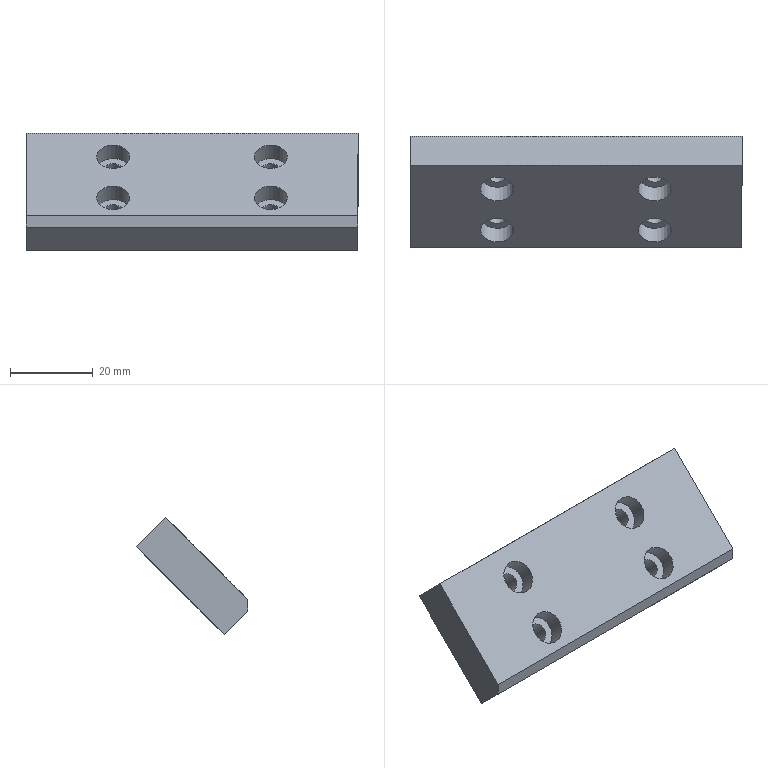Component | SolidWorks | ClampingArm2-1_A27-1 | 1 solid | 27 faces | box 80 x 26.88 x 28.28 mm | volume 22572 mm3 | cylinder 16 | plane 11 | commonest cylinder face diameters 8 x8 4.5 x8 | material Urethane
build123d program:
from build123d import *

# Parameters (mm, degrees)
SKETCH1_W                                          = 80
SKETCH1_H                                          = 30
BOSS_EXTRUDE1_DEPTH                                = 5
HOLE_SIZE_ACCORDING_TO_TYPE_1_OF_HEXAG_D           = 4.5
HOLE_SIZE_ACCORDING_TO_TYPE_1_OF_HEXAG_CBORE_D     = 8
HOLE_SIZE_ACCORDING_TO_TYPE_1_OF_HEXAG_CBORE_DEPTH = 4.6
CHAMFER1_SIZE                                      = 2


with BuildPart() as part:
    # Sketch1 → Boss-Extrude1 (new, symmetric)
    with BuildSketch(Plane(origin=(0, 0, 0), x_dir=(0, 0, -1), z_dir=(1, 0, 0))):
        Rectangle(SKETCH1_W, SKETCH1_H)
    extrude(amount=BOSS_EXTRUDE1_DEPTH, both=True)

    # Hole Size _According to_ Type 1 of Hexag (through all)
    with Locations(Plane(origin=(5, 0, 0), x_dir=(0, 0, -1), z_dir=(1, 0, 0))):
        with Locations((-19, 7), (-19, -7), (19, -7), (19, 7)):
            CounterBoreHole(HOLE_SIZE_ACCORDING_TO_TYPE_1_OF_HEXAG_D / 2, HOLE_SIZE_ACCORDING_TO_TYPE_1_OF_HEXAG_CBORE_D / 2, HOLE_SIZE_ACCORDING_TO_TYPE_1_OF_HEXAG_CBORE_DEPTH)

    # Chamfer1
    chamfer1_edges = [part.edges().sort_by_distance(p)[0] for p in [
        (5, 15, 0),
    ]]
    chamfer(chamfer1_edges, length=CHAMFER1_SIZE)


solid = part.part

# Placed as in the assembly
solid = solid.moved(Location((-43.051, 50.356, -166.066), (-135.019, 90, 0)))
STEP:
#1=CARTESIAN_POINT('',(-0.7894,1.776,-6.722));
#2=VERTEX_POINT('',#1);
#3=CARTESIAN_POINT('',(-1.104,1.776,-6.722));
#4=VERTEX_POINT('',#3);
#5=CARTESIAN_POINT('',(-0.9469,1.776,-6.722));
#6=DIRECTION('',(-0.,-0.7069,0.7073));
#7=DIRECTION('',(-1.,0.,0.));
#8=AXIS2_PLACEMENT_3D('',#5,#6,#7);
#9=CIRCLE('',#8,0.1575);
#10=EDGE_CURVE('',#2,#4,#9,.T.);
#11=ORIENTED_EDGE('',*,*,#10,.F.);
#12=CARTESIAN_POINT('',(-0.7894,1.648,-6.594));
#13=VERTEX_POINT('',#12);
#14=CARTESIAN_POINT('',(-0.7894,1.648,-6.594));
#15=DIRECTION('',(-0.,-0.7069,0.7073));
#16=VECTOR('',#15,39.37);
#17=LINE('',#14,#16);
#18=EDGE_CURVE('',#2,#13,#17,.T.);
#19=ORIENTED_EDGE('',*,*,#18,.T.);
#20=CARTESIAN_POINT('',(-1.104,1.648,-6.594));
#21=VERTEX_POINT('',#20);
#22=CARTESIAN_POINT('',(-0.9469,1.648,-6.594));
#23=DIRECTION('',(-0.,-0.7069,0.7073));
#24=DIRECTION('',(-1.,0.,0.));
#25=AXIS2_PLACEMENT_3D('',#22,#23,#24);
#26=CIRCLE('',#25,0.1575);
#27=EDGE_CURVE('',#13,#21,#26,.T.);
#28=ORIENTED_EDGE('',*,*,#27,.T.);
#29=CARTESIAN_POINT('',(-1.104,1.648,-6.594));
#30=DIRECTION('',(-0.,-0.7069,0.7073));
#31=VECTOR('',#30,39.37);
#32=LINE('',#29,#31);
#33=EDGE_CURVE('',#4,#21,#32,.T.);
#34=ORIENTED_EDGE('',*,*,#33,.F.);
#35=EDGE_LOOP('',(#11,#19,#28,#34));
#36=FACE_OUTER_BOUND('',#35,.T.);
#37=CARTESIAN_POINT('',(-0.9469,1.648,-6.594));
#38=DIRECTION('',(-0.,-0.7069,0.7073));
#39=DIRECTION('',(-1.,0.,0.));
#40=AXIS2_PLACEMENT_3D('',#37,#38,#39);
#41=CYLINDRICAL_SURFACE('',#40,0.1575);
#42=ADVANCED_FACE('',(#36),#41,.F.);
#43=CARTESIAN_POINT('',(-0.8583,1.927,-6.872));
#44=VERTEX_POINT('',#43);
#45=CARTESIAN_POINT('',(-1.035,1.927,-6.872));
#46=VERTEX_POINT('',#45);
#47=CARTESIAN_POINT('',(-0.9469,1.927,-6.872));
#48=DIRECTION('',(-0.,-0.7069,0.7073));
#49=DIRECTION('',(-1.,0.,0.));
#50=AXIS2_PLACEMENT_3D('',#47,#48,#49);
#51=CIRCLE('',#50,0.08858);
#52=EDGE_CURVE('',#44,#46,#51,.T.);
#53=ORIENTED_EDGE('',*,*,#52,.F.);
#54=CARTESIAN_POINT('',(-0.8583,1.776,-6.722));
#55=VERTEX_POINT('',#54);
#56=CARTESIAN_POINT('',(-0.8583,1.648,-6.594));
#57=DIRECTION('',(-0.,-0.7069,0.7073));
#58=VECTOR('',#57,39.37);
#59=LINE('',#56,#58);
#60=EDGE_CURVE('',#44,#55,#59,.T.);
#61=ORIENTED_EDGE('',*,*,#60,.T.);
#62=CARTESIAN_POINT('',(-1.035,1.776,-6.722));
#63=VERTEX_POINT('',#62);
#64=CARTESIAN_POINT('',(-0.9469,1.776,-6.722));
#65=DIRECTION('',(-0.,-0.7069,0.7073));
#66=DIRECTION('',(-1.,0.,0.));
#67=AXIS2_PLACEMENT_3D('',#64,#65,#66);
#68=CIRCLE('',#67,0.08858);
#69=EDGE_CURVE('',#55,#63,#68,.T.);
#70=ORIENTED_EDGE('',*,*,#69,.T.);
#71=CARTESIAN_POINT('',(-1.035,1.648,-6.594));
#72=DIRECTION('',(-0.,-0.7069,0.7073));
#73=VECTOR('',#72,39.37);
#74=LINE('',#71,#73);
#75=EDGE_CURVE('',#46,#63,#74,.T.);
#76=ORIENTED_EDGE('',*,*,#75,.F.);
#77=EDGE_LOOP('',(#53,#61,#70,#76));
#78=FACE_OUTER_BOUND('',#77,.T.);
#79=CARTESIAN_POINT('',(-0.9469,1.648,-6.594));
#80=DIRECTION('',(-0.,-0.7069,0.7073));
#81=DIRECTION('',(-1.,0.,0.));
#82=AXIS2_PLACEMENT_3D('',#79,#80,#81);
#83=CYLINDRICAL_SURFACE('',#82,0.08858);
#84=ADVANCED_FACE('',(#78),#83,.F.);
#85=CARTESIAN_POINT('',(-0.7894,2.166,-6.332));
#86=VERTEX_POINT('',#85);
#87=CARTESIAN_POINT('',(-1.104,2.166,-6.332));
#88=VERTEX_POINT('',#87);
#89=CARTESIAN_POINT('',(-0.9469,2.166,-6.332));
#90=DIRECTION('',(-0.,-0.7069,0.7073));
#91=DIRECTION('',(-1.,0.,0.));
#92=AXIS2_PLACEMENT_3D('',#89,#90,#91);
#93=CIRCLE('',#92,0.1575);
#94=EDGE_CURVE('',#86,#88,#93,.T.);
#95=ORIENTED_EDGE('',*,*,#94,.F.);
#96=CARTESIAN_POINT('',(-0.7894,2.038,-6.204));
#97=VERTEX_POINT('',#96);
#98=CARTESIAN_POINT('',(-0.7894,2.038,-6.204));
#99=DIRECTION('',(-0.,-0.7069,0.7073));
#100=VECTOR('',#99,39.37);
#101=LINE('',#98,#100);
#102=EDGE_CURVE('',#86,#97,#101,.T.);
#103=ORIENTED_EDGE('',*,*,#102,.T.);
#104=CARTESIAN_POINT('',(-1.104,2.038,-6.204));
#105=VERTEX_POINT('',#104);
#106=CARTESIAN_POINT('',(-0.9469,2.038,-6.204));
#107=DIRECTION('',(-0.,-0.7069,0.7073));
#108=DIRECTION('',(-1.,0.,0.));
#109=AXIS2_PLACEMENT_3D('',#106,#107,#108);
#110=CIRCLE('',#109,0.1575);
#111=EDGE_CURVE('',#97,#105,#110,.T.);
#112=ORIENTED_EDGE('',*,*,#111,.T.);
#113=CARTESIAN_POINT('',(-1.104,2.038,-6.204));
#114=DIRECTION('',(-0.,-0.7069,0.7073));
#115=VECTOR('',#114,39.37);
#116=LINE('',#113,#115);
#117=EDGE_CURVE('',#88,#105,#116,.T.);
#118=ORIENTED_EDGE('',*,*,#117,.F.);
#119=EDGE_LOOP('',(#95,#103,#112,#118));
#120=FACE_OUTER_BOUND('',#119,.T.);
#121=CARTESIAN_POINT('',(-0.9469,2.038,-6.204));
#122=DIRECTION('',(-0.,-0.7069,0.7073));
#123=DIRECTION('',(-1.,0.,0.));
#124=AXIS2_PLACEMENT_3D('',#121,#122,#123);
#125=CYLINDRICAL_SURFACE('',#124,0.1575);
#126=ADVANCED_FACE('',(#120),#125,.F.);
#127=CARTESIAN_POINT('',(-0.8583,2.317,-6.482));
#128=VERTEX_POINT('',#127);
#129=CARTESIAN_POINT('',(-1.035,2.317,-6.482));
#130=VERTEX_POINT('',#129);
#131=CARTESIAN_POINT('',(-0.9469,2.317,-6.482));
#132=DIRECTION('',(-0.,-0.7069,0.7073));
#133=DIRECTION('',(-1.,0.,0.));
#134=AXIS2_PLACEMENT_3D('',#131,#132,#133);
#135=CIRCLE('',#134,0.08858);
#136=EDGE_CURVE('',#128,#130,#135,.T.);
#137=ORIENTED_EDGE('',*,*,#136,.F.);
#138=CARTESIAN_POINT('',(-0.8583,2.166,-6.332));
#139=VERTEX_POINT('',#138);
#140=CARTESIAN_POINT('',(-0.8583,2.038,-6.204));
#141=DIRECTION('',(-0.,-0.7069,0.7073));
#142=VECTOR('',#141,39.37);
#143=LINE('',#140,#142);
#144=EDGE_CURVE('',#128,#139,#143,.T.);
#145=ORIENTED_EDGE('',*,*,#144,.T.);
#146=CARTESIAN_POINT('',(-1.035,2.166,-6.332));
#147=VERTEX_POINT('',#146);
#148=CARTESIAN_POINT('',(-0.9469,2.166,-6.332));
#149=DIRECTION('',(-0.,-0.7069,0.7073));
#150=DIRECTION('',(-1.,0.,0.));
#151=AXIS2_PLACEMENT_3D('',#148,#149,#150);
#152=CIRCLE('',#151,0.08858);
#153=EDGE_CURVE('',#139,#147,#152,.T.);
#154=ORIENTED_EDGE('',*,*,#153,.T.);
#155=CARTESIAN_POINT('',(-1.035,2.038,-6.204));
#156=DIRECTION('',(-0.,-0.7069,0.7073));
#157=VECTOR('',#156,39.37);
#158=LINE('',#155,#157);
#159=EDGE_CURVE('',#130,#147,#158,.T.);
#160=ORIENTED_EDGE('',*,*,#159,.F.);
#161=EDGE_LOOP('',(#137,#145,#154,#160));
#162=FACE_OUTER_BOUND('',#161,.T.);
#163=CARTESIAN_POINT('',(-0.9469,2.038,-6.204));
#164=DIRECTION('',(-0.,-0.7069,0.7073));
#165=DIRECTION('',(-1.,0.,0.));
#166=AXIS2_PLACEMENT_3D('',#163,#164,#165);
#167=CYLINDRICAL_SURFACE('',#166,0.08858);
#168=ADVANCED_FACE('',(#162),#167,.F.);
#169=CARTESIAN_POINT('',(-2.285,2.166,-6.332));
#170=VERTEX_POINT('',#169);
#171=CARTESIAN_POINT('',(-2.6,2.166,-6.332));
#172=VERTEX_POINT('',#171);
#173=CARTESIAN_POINT('',(-2.443,2.166,-6.332));
#174=DIRECTION('',(-0.,-0.7069,0.7073));
#175=DIRECTION('',(-1.,0.,0.));
#176=AXIS2_PLACEMENT_3D('',#173,#174,#175);
#177=CIRCLE('',#176,0.1575);
#178=EDGE_CURVE('',#170,#172,#177,.T.);
#179=ORIENTED_EDGE('',*,*,#178,.F.);
#180=CARTESIAN_POINT('',(-2.285,2.038,-6.204));
#181=VERTEX_POINT('',#180);
#182=CARTESIAN_POINT('',(-2.285,2.038,-6.204));
#183=DIRECTION('',(-0.,-0.7069,0.7073));
#184=VECTOR('',#183,39.37);
#185=LINE('',#182,#184);
#186=EDGE_CURVE('',#170,#181,#185,.T.);
#187=ORIENTED_EDGE('',*,*,#186,.T.);
#188=CARTESIAN_POINT('',(-2.6,2.038,-6.204));
#189=VERTEX_POINT('',#188);
#190=CARTESIAN_POINT('',(-2.443,2.038,-6.204));
#191=DIRECTION('',(-0.,-0.7069,0.7073));
#192=DIRECTION('',(-1.,0.,0.));
#193=AXIS2_PLACEMENT_3D('',#190,#191,#192);
#194=CIRCLE('',#193,0.1575);
#195=EDGE_CURVE('',#181,#189,#194,.T.);
#196=ORIENTED_EDGE('',*,*,#195,.T.);
#197=CARTESIAN_POINT('',(-2.6,2.038,-6.204));
#198=DIRECTION('',(-0.,-0.7069,0.7073));
#199=VECTOR('',#198,39.37);
#200=LINE('',#197,#199);
#201=EDGE_CURVE('',#172,#189,#200,.T.);
#202=ORIENTED_EDGE('',*,*,#201,.F.);
#203=EDGE_LOOP('',(#179,#187,#196,#202));
#204=FACE_OUTER_BOUND('',#203,.T.);
#205=CARTESIAN_POINT('',(-2.443,2.038,-6.204));
#206=DIRECTION('',(-0.,-0.7069,0.7073));
#207=DIRECTION('',(-1.,0.,0.));
#208=AXIS2_PLACEMENT_3D('',#205,#206,#207);
#209=CYLINDRICAL_SURFACE('',#208,0.1575);
#210=ADVANCED_FACE('',(#204),#209,.F.);
#211=CARTESIAN_POINT('',(-2.354,2.317,-6.482));
#212=VERTEX_POINT('',#211);
#213=CARTESIAN_POINT('',(-2.532,2.317,-6.482));
#214=VERTEX_POINT('',#213);
#215=CARTESIAN_POINT('',(-2.443,2.317,-6.482));
#216=DIRECTION('',(-0.,-0.7069,0.7073));
#217=DIRECTION('',(-1.,0.,0.));
#218=AXIS2_PLACEMENT_3D('',#215,#216,#217);
#219=CIRCLE('',#218,0.08858);
#220=EDGE_CURVE('',#212,#214,#219,.T.);
#221=ORIENTED_EDGE('',*,*,#220,.F.);
#222=CARTESIAN_POINT('',(-2.354,2.166,-6.332));
#223=VERTEX_POINT('',#222);
#224=CARTESIAN_POINT('',(-2.354,2.038,-6.204));
#225=DIRECTION('',(-0.,-0.7069,0.7073));
#226=VECTOR('',#225,39.37);
#227=LINE('',#224,#226);
#228=EDGE_CURVE('',#212,#223,#227,.T.);
#229=ORIENTED_EDGE('',*,*,#228,.T.);
#230=CARTESIAN_POINT('',(-2.532,2.166,-6.332));
#231=VERTEX_POINT('',#230);
#232=CARTESIAN_POINT('',(-2.443,2.166,-6.332));
#233=DIRECTION('',(-0.,-0.7069,0.7073));
#234=DIRECTION('',(-1.,0.,0.));
#235=AXIS2_PLACEMENT_3D('',#232,#233,#234);
#236=CIRCLE('',#235,0.08858);
#237=EDGE_CURVE('',#223,#231,#236,.T.);
#238=ORIENTED_EDGE('',*,*,#237,.T.);
#239=CARTESIAN_POINT('',(-2.532,2.038,-6.204));
#240=DIRECTION('',(-0.,-0.7069,0.7073));
#241=VECTOR('',#240,39.37);
#242=LINE('',#239,#241);
#243=EDGE_CURVE('',#214,#231,#242,.T.);
#244=ORIENTED_EDGE('',*,*,#243,.F.);
#245=EDGE_LOOP('',(#221,#229,#238,#244));
#246=FACE_OUTER_BOUND('',#245,.T.);
#247=CARTESIAN_POINT('',(-2.443,2.038,-6.204));
#248=DIRECTION('',(-0.,-0.7069,0.7073));
#249=DIRECTION('',(-1.,0.,0.));
#250=AXIS2_PLACEMENT_3D('',#247,#248,#249);
#251=CYLINDRICAL_SURFACE('',#250,0.08858);
#252=ADVANCED_FACE('',(#246),#251,.F.);
#253=CARTESIAN_POINT('',(-2.285,1.776,-6.722));
#254=VERTEX_POINT('',#253);
#255=CARTESIAN_POINT('',(-2.6,1.776,-6.722));
#256=VERTEX_POINT('',#255);
#257=CARTESIAN_POINT('',(-2.443,1.776,-6.722));
#258=DIRECTION('',(-0.,-0.7069,0.7073));
#259=DIRECTION('',(-1.,0.,0.));
#260=AXIS2_PLACEMENT_3D('',#257,#258,#259);
#261=CIRCLE('',#260,0.1575);
#262=EDGE_CURVE('',#254,#256,#261,.T.);
#263=ORIENTED_EDGE('',*,*,#262,.F.);
#264=CARTESIAN_POINT('',(-2.285,1.648,-6.594));
#265=VERTEX_POINT('',#264);
#266=CARTESIAN_POINT('',(-2.285,1.648,-6.594));
#267=DIRECTION('',(-0.,-0.7069,0.7073));
#268=VECTOR('',#267,39.37);
#269=LINE('',#266,#268);
#270=EDGE_CURVE('',#254,#265,#269,.T.);
#271=ORIENTED_EDGE('',*,*,#270,.T.);
#272=CARTESIAN_POINT('',(-2.6,1.648,-6.594));
#273=VERTEX_POINT('',#272);
#274=CARTESIAN_POINT('',(-2.443,1.648,-6.594));
#275=DIRECTION('',(-0.,-0.7069,0.7073));
#276=DIRECTION('',(-1.,0.,0.));
#277=AXIS2_PLACEMENT_3D('',#274,#275,#276);
#278=CIRCLE('',#277,0.1575);
#279=EDGE_CURVE('',#265,#273,#278,.T.);
#280=ORIENTED_EDGE('',*,*,#279,.T.);
#281=CARTESIAN_POINT('',(-2.6,1.648,-6.594));
#282=DIRECTION('',(-0.,-0.7069,0.7073));
#283=VECTOR('',#282,39.37);
#284=LINE('',#281,#283);
#285=EDGE_CURVE('',#256,#273,#284,.T.);
#286=ORIENTED_EDGE('',*,*,#285,.F.);
#287=EDGE_LOOP('',(#263,#271,#280,#286));
#288=FACE_OUTER_BOUND('',#287,.T.);
#289=CARTESIAN_POINT('',(-2.443,1.648,-6.594));
#290=DIRECTION('',(-0.,-0.7069,0.7073));
#291=DIRECTION('',(-1.,0.,0.));
#292=AXIS2_PLACEMENT_3D('',#289,#290,#291);
#293=CYLINDRICAL_SURFACE('',#292,0.1575);
#294=ADVANCED_FACE('',(#288),#293,.F.);
#295=CARTESIAN_POINT('',(-2.354,1.927,-6.872));
#296=VERTEX_POINT('',#295);
#297=CARTESIAN_POINT('',(-2.532,1.927,-6.872));
#298=VERTEX_POINT('',#297);
#299=CARTESIAN_POINT('',(-2.443,1.927,-6.872));
#300=DIRECTION('',(-0.,-0.7069,0.7073));
#301=DIRECTION('',(-1.,0.,0.));
#302=AXIS2_PLACEMENT_3D('',#299,#300,#301);
#303=CIRCLE('',#302,0.08858);
#304=EDGE_CURVE('',#296,#298,#303,.T.);
#305=ORIENTED_EDGE('',*,*,#304,.F.);
#306=CARTESIAN_POINT('',(-2.354,1.776,-6.722));
#307=VERTEX_POINT('',#306);
#308=CARTESIAN_POINT('',(-2.354,1.648,-6.594));
#309=DIRECTION('',(-0.,-0.7069,0.7073));
#310=VECTOR('',#309,39.37);
#311=LINE('',#308,#310);
#312=EDGE_CURVE('',#296,#307,#311,.T.);
#313=ORIENTED_EDGE('',*,*,#312,.T.);
#314=CARTESIAN_POINT('',(-2.532,1.776,-6.722));
#315=VERTEX_POINT('',#314);
#316=CARTESIAN_POINT('',(-2.443,1.776,-6.722));
#317=DIRECTION('',(-0.,-0.7069,0.7073));
#318=DIRECTION('',(-1.,0.,0.));
#319=AXIS2_PLACEMENT_3D('',#316,#317,#318);
#320=CIRCLE('',#319,0.08858);
#321=EDGE_CURVE('',#307,#315,#320,.T.);
#322=ORIENTED_EDGE('',*,*,#321,.T.);
#323=CARTESIAN_POINT('',(-2.532,1.648,-6.594));
#324=DIRECTION('',(-0.,-0.7069,0.7073));
#325=VECTOR('',#324,39.37);
#326=LINE('',#323,#325);
#327=EDGE_CURVE('',#298,#315,#326,.T.);
#328=ORIENTED_EDGE('',*,*,#327,.F.);
#329=EDGE_LOOP('',(#305,#313,#322,#328));
#330=FACE_OUTER_BOUND('',#329,.T.);
#331=CARTESIAN_POINT('',(-2.443,1.648,-6.594));
#332=DIRECTION('',(-0.,-0.7069,0.7073));
#333=DIRECTION('',(-1.,0.,0.));
#334=AXIS2_PLACEMENT_3D('',#331,#332,#333);
#335=CYLINDRICAL_SURFACE('',#334,0.08858);
#336=ADVANCED_FACE('',(#330),#335,.F.);
#337=CARTESIAN_POINT('',(-3.27,1.481,-6.872));
#338=VERTEX_POINT('',#337);
#339=CARTESIAN_POINT('',(-3.27,1.704,-7.095));
#340=VERTEX_POINT('',#339);
#341=CARTESIAN_POINT('',(-3.27,1.426,-6.816));
#342=DIRECTION('',(0.,0.7069,-0.7073));
#343=VECTOR('',#342,39.37);
#344=LINE('',#341,#343);
#345=EDGE_CURVE('',#338,#340,#344,.T.);
#346=ORIENTED_EDGE('',*,*,#345,.F.);
#347=CARTESIAN_POINT('',(-3.27,1.481,-6.761));
#348=VERTEX_POINT('',#347);
#349=CARTESIAN_POINT('',(-3.27,1.481,-6.761));
#350=DIRECTION('',(0.,0.0003333,1.));
#351=VECTOR('',#350,39.37);
#352=LINE('',#349,#351);
#353=EDGE_CURVE('',#338,#348,#352,.T.);
#354=ORIENTED_EDGE('',*,*,#353,.T.);
#355=CARTESIAN_POINT('',(-3.27,2.261,-5.981));
#356=VERTEX_POINT('',#355);
#357=CARTESIAN_POINT('',(-3.27,1.426,-6.816));
#358=DIRECTION('',(-0.,-0.7073,-0.7069));
#359=VECTOR('',#358,39.37);
#360=LINE('',#357,#359);
#361=EDGE_CURVE('',#356,#348,#360,.T.);
#362=ORIENTED_EDGE('',*,*,#361,.F.);
#363=CARTESIAN_POINT('',(-3.27,2.539,-6.26));
#364=VERTEX_POINT('',#363);
#365=CARTESIAN_POINT('',(-3.27,2.261,-5.981));
#366=DIRECTION('',(0.,0.7069,-0.7073));
#367=VECTOR('',#366,39.37);
#368=LINE('',#365,#367);
#369=EDGE_CURVE('',#356,#364,#368,.T.);
#370=ORIENTED_EDGE('',*,*,#369,.T.);
#371=CARTESIAN_POINT('',(-3.27,1.704,-7.095));
#372=DIRECTION('',(-0.,-0.7073,-0.7069));
#373=VECTOR('',#372,39.37);
#374=LINE('',#371,#373);
#375=EDGE_CURVE('',#364,#340,#374,.T.);
#376=ORIENTED_EDGE('',*,*,#375,.T.);
#377=EDGE_LOOP('',(#346,#354,#362,#370,#376));
#378=FACE_OUTER_BOUND('',#377,.T.);
#379=CARTESIAN_POINT('',(-3.27,1.426,-6.816));
#380=DIRECTION('',(1.,-0.,-0.));
#381=DIRECTION('',(0.,0.7073,0.7069));
#382=AXIS2_PLACEMENT_3D('',#379,#380,#381);
#383=PLANE('',#382);
#384=ADVANCED_FACE('',(#378),#383,.F.);
#385=CARTESIAN_POINT('',(-0.1201,1.481,-6.872));
#386=VERTEX_POINT('',#385);
#387=CARTESIAN_POINT('',(-0.1201,1.704,-7.095));
#388=VERTEX_POINT('',#387);
#389=CARTESIAN_POINT('',(-0.1201,1.426,-6.816));
#390=DIRECTION('',(0.,0.7069,-0.7073));
#391=VECTOR('',#390,39.37);
#392=LINE('',#389,#391);
#393=EDGE_CURVE('',#386,#388,#392,.T.);
#394=ORIENTED_EDGE('',*,*,#393,.F.);
#395=CARTESIAN_POINT('',(-3.27,1.481,-6.872));
#396=DIRECTION('',(-1.,0.,0.));
#397=VECTOR('',#396,39.37);
#398=LINE('',#395,#397);
#399=EDGE_CURVE('',#386,#338,#398,.T.);
#400=ORIENTED_EDGE('',*,*,#399,.T.);
#401=ORIENTED_EDGE('',*,*,#345,.T.);
#402=CARTESIAN_POINT('',(-0.1201,1.704,-7.095));
#403=DIRECTION('',(1.,-0.,-0.));
#404=VECTOR('',#403,39.37);
#405=LINE('',#402,#404);
#406=EDGE_CURVE('',#340,#388,#405,.T.);
#407=ORIENTED_EDGE('',*,*,#406,.T.);
#408=EDGE_LOOP('',(#394,#400,#401,#407));
#409=FACE_OUTER_BOUND('',#408,.T.);
#410=CARTESIAN_POINT('',(-0.1201,1.426,-6.816));
#411=DIRECTION('',(0.,0.7073,0.7069));
#412=DIRECTION('',(-1.,0.,0.));
#413=AXIS2_PLACEMENT_3D('',#410,#411,#412);
#414=PLANE('',#413);
#415=ADVANCED_FACE('',(#409),#414,.F.);
#416=CARTESIAN_POINT('',(-0.1201,1.481,-6.761));
#417=VERTEX_POINT('',#416);
#418=CARTESIAN_POINT('',(-0.1201,2.261,-5.981));
#419=VERTEX_POINT('',#418);
#420=CARTESIAN_POINT('',(-0.1201,1.426,-6.816));
#421=DIRECTION('',(0.,0.7073,0.7069));
#422=VECTOR('',#421,39.37);
#423=LINE('',#420,#422);
#424=EDGE_CURVE('',#417,#419,#423,.T.);
#425=ORIENTED_EDGE('',*,*,#424,.F.);
#426=CARTESIAN_POINT('',(-0.1201,1.481,-6.761));
#427=DIRECTION('',(-0.,-0.0003333,-1.));
#428=VECTOR('',#427,39.37);
#429=LINE('',#426,#428);
#430=EDGE_CURVE('',#417,#386,#429,.T.);
#431=ORIENTED_EDGE('',*,*,#430,.T.);
#432=ORIENTED_EDGE('',*,*,#393,.T.);
#433=CARTESIAN_POINT('',(-0.1201,2.539,-6.26));
#434=VERTEX_POINT('',#433);
#435=CARTESIAN_POINT('',(-0.1201,1.704,-7.095));
#436=DIRECTION('',(0.,0.7073,0.7069));
#437=VECTOR('',#436,39.37);
#438=LINE('',#435,#437);
#439=EDGE_CURVE('',#388,#434,#438,.T.);
#440=ORIENTED_EDGE('',*,*,#439,.T.);
#441=CARTESIAN_POINT('',(-0.1201,2.261,-5.981));
#442=DIRECTION('',(0.,0.7069,-0.7073));
#443=VECTOR('',#442,39.37);
#444=LINE('',#441,#443);
#445=EDGE_CURVE('',#419,#434,#444,.T.);
#446=ORIENTED_EDGE('',*,*,#445,.F.);
#447=EDGE_LOOP('',(#425,#431,#432,#440,#446));
#448=FACE_OUTER_BOUND('',#447,.T.);
#449=CARTESIAN_POINT('',(-0.1201,1.426,-6.816));
#450=DIRECTION('',(-1.,0.,0.));
#451=DIRECTION('',(0.,0.7069,-0.7073));
#452=AXIS2_PLACEMENT_3D('',#449,#450,#451);
#453=PLANE('',#452);
#454=ADVANCED_FACE('',(#448),#453,.F.);
#455=CARTESIAN_POINT('',(-0.1201,2.539,-6.26));
#456=DIRECTION('',(-1.,0.,0.));
#457=VECTOR('',#456,39.37);
#458=LINE('',#455,#457);
#459=EDGE_CURVE('',#434,#364,#458,.T.);
#460=ORIENTED_EDGE('',*,*,#459,.T.);
#461=ORIENTED_EDGE('',*,*,#369,.F.);
#462=CARTESIAN_POINT('',(-0.1201,2.261,-5.981));
#463=DIRECTION('',(-1.,0.,0.));
#464=VECTOR('',#463,39.37);
#465=LINE('',#462,#464);
#466=EDGE_CURVE('',#419,#356,#465,.T.);
#467=ORIENTED_EDGE('',*,*,#466,.F.);
#468=ORIENTED_EDGE('',*,*,#445,.T.);
#469=EDGE_LOOP('',(#460,#461,#467,#468));
#470=FACE_OUTER_BOUND('',#469,.T.);
#471=CARTESIAN_POINT('',(-0.1201,2.261,-5.981));
#472=DIRECTION('',(-0.,-0.7073,-0.7069));
#473=DIRECTION('',(1.,-0.,-0.));
#474=AXIS2_PLACEMENT_3D('',#471,#472,#473);
#475=PLANE('',#474);
#476=ADVANCED_FACE('',(#470),#475,.F.);
#477=CARTESIAN_POINT('',(-0.9469,1.648,-6.594));
#478=DIRECTION('',(-0.,-0.7069,0.7073));
#479=DIRECTION('',(-1.,0.,0.));
#480=AXIS2_PLACEMENT_3D('',#477,#478,#479);
#481=CIRCLE('',#480,0.1575);
#482=EDGE_CURVE('',#21,#13,#481,.T.);
#483=ORIENTED_EDGE('',*,*,#482,.F.);
#484=ORIENTED_EDGE('',*,*,#27,.F.);
#485=EDGE_LOOP('',(#483,#484));
#486=FACE_BOUND('',#485,.T.);
#487=CARTESIAN_POINT('',(-0.9469,2.038,-6.204));
#488=DIRECTION('',(-0.,-0.7069,0.7073));
#489=DIRECTION('',(-1.,0.,0.));
#490=AXIS2_PLACEMENT_3D('',#487,#488,#489);
#491=CIRCLE('',#490,0.1575);
#492=EDGE_CURVE('',#105,#97,#491,.T.);
#493=ORIENTED_EDGE('',*,*,#492,.F.);
#494=ORIENTED_EDGE('',*,*,#111,.F.);
#495=EDGE_LOOP('',(#493,#494));
#496=FACE_BOUND('',#495,.T.);
#497=CARTESIAN_POINT('',(-2.443,2.038,-6.204));
#498=DIRECTION('',(-0.,-0.7069,0.7073));
#499=DIRECTION('',(-1.,0.,0.));
#500=AXIS2_PLACEMENT_3D('',#497,#498,#499);
#501=CIRCLE('',#500,0.1575);
#502=EDGE_CURVE('',#189,#181,#501,.T.);
#503=ORIENTED_EDGE('',*,*,#502,.F.);
#504=ORIENTED_EDGE('',*,*,#195,.F.);
#505=EDGE_LOOP('',(#503,#504));
#506=FACE_BOUND('',#505,.T.);
#507=CARTESIAN_POINT('',(-2.443,1.648,-6.594));
#508=DIRECTION('',(-0.,-0.7069,0.7073));
#509=DIRECTION('',(-1.,0.,0.));
#510=AXIS2_PLACEMENT_3D('',#507,#508,#509);
#511=CIRCLE('',#510,0.1575);
#512=EDGE_CURVE('',#273,#265,#511,.T.);
#513=ORIENTED_EDGE('',*,*,#512,.F.);
#514=ORIENTED_EDGE('',*,*,#279,.F.);
#515=EDGE_LOOP('',(#513,#514));
#516=FACE_BOUND('',#515,.T.);
#517=ORIENTED_EDGE('',*,*,#361,.T.);
#518=CARTESIAN_POINT('',(-0.1201,1.481,-6.761));
#519=DIRECTION('',(1.,-0.,-0.));
#520=VECTOR('',#519,39.37);
#521=LINE('',#518,#520);
#522=EDGE_CURVE('',#348,#417,#521,.T.);
#523=ORIENTED_EDGE('',*,*,#522,.T.);
#524=ORIENTED_EDGE('',*,*,#424,.T.);
#525=ORIENTED_EDGE('',*,*,#466,.T.);
#526=EDGE_LOOP('',(#517,#523,#524,#525));
#527=FACE_OUTER_BOUND('',#526,.T.);
#528=CARTESIAN_POINT('',(-1.695,1.843,-6.399));
#529=DIRECTION('',(-0.,-0.7069,0.7073));
#530=DIRECTION('',(-1.,0.,0.));
#531=AXIS2_PLACEMENT_3D('',#528,#529,#530);
#532=PLANE('',#531);
#533=ADVANCED_FACE('',(#486,#496,#506,#516,#527),#532,.T.);
#534=CARTESIAN_POINT('',(-0.9469,1.927,-6.872));
#535=DIRECTION('',(-0.,-0.7069,0.7073));
#536=DIRECTION('',(-1.,0.,0.));
#537=AXIS2_PLACEMENT_3D('',#534,#535,#536);
#538=CIRCLE('',#537,0.08858);
#539=EDGE_CURVE('',#46,#44,#538,.T.);
#540=ORIENTED_EDGE('',*,*,#539,.T.);
#541=ORIENTED_EDGE('',*,*,#52,.T.);
#542=EDGE_LOOP('',(#540,#541));
#543=FACE_BOUND('',#542,.T.);
#544=CARTESIAN_POINT('',(-0.9469,2.317,-6.482));
#545=DIRECTION('',(-0.,-0.7069,0.7073));
#546=DIRECTION('',(-1.,0.,0.));
#547=AXIS2_PLACEMENT_3D('',#544,#545,#546);
#548=CIRCLE('',#547,0.08858);
#549=EDGE_CURVE('',#130,#128,#548,.T.);
#550=ORIENTED_EDGE('',*,*,#549,.T.);
#551=ORIENTED_EDGE('',*,*,#136,.T.);
#552=EDGE_LOOP('',(#550,#551));
#553=FACE_BOUND('',#552,.T.);
#554=CARTESIAN_POINT('',(-2.443,2.317,-6.482));
#555=DIRECTION('',(-0.,-0.7069,0.7073));
#556=DIRECTION('',(-1.,0.,0.));
#557=AXIS2_PLACEMENT_3D('',#554,#555,#556);
#558=CIRCLE('',#557,0.08858);
#559=EDGE_CURVE('',#214,#212,#558,.T.);
#560=ORIENTED_EDGE('',*,*,#559,.T.);
#561=ORIENTED_EDGE('',*,*,#220,.T.);
#562=EDGE_LOOP('',(#560,#561));
#563=FACE_BOUND('',#562,.T.);
#564=CARTESIAN_POINT('',(-2.443,1.927,-6.872));
#565=DIRECTION('',(-0.,-0.7069,0.7073));
#566=DIRECTION('',(-1.,0.,0.));
#567=AXIS2_PLACEMENT_3D('',#564,#565,#566);
#568=CIRCLE('',#567,0.08858);
#569=EDGE_CURVE('',#298,#296,#568,.T.);
#570=ORIENTED_EDGE('',*,*,#569,.T.);
#571=ORIENTED_EDGE('',*,*,#304,.T.);
#572=EDGE_LOOP('',(#570,#571));
#573=FACE_BOUND('',#572,.T.);
#574=ORIENTED_EDGE('',*,*,#375,.F.);
#575=ORIENTED_EDGE('',*,*,#459,.F.);
#576=ORIENTED_EDGE('',*,*,#439,.F.);
#577=ORIENTED_EDGE('',*,*,#406,.F.);
#578=EDGE_LOOP('',(#574,#575,#576,#577));
#579=FACE_OUTER_BOUND('',#578,.T.);
#580=CARTESIAN_POINT('',(-1.695,2.122,-6.677));
#581=DIRECTION('',(-0.,-0.7069,0.7073));
#582=DIRECTION('',(-1.,0.,0.));
#583=AXIS2_PLACEMENT_3D('',#580,#581,#582);
#584=PLANE('',#583);
#585=ADVANCED_FACE('',(#543,#553,#563,#573,#579),#584,.F.);
#586=ORIENTED_EDGE('',*,*,#312,.F.);
#587=ORIENTED_EDGE('',*,*,#569,.F.);
#588=ORIENTED_EDGE('',*,*,#327,.T.);
#589=CARTESIAN_POINT('',(-2.443,1.776,-6.722));
#590=DIRECTION('',(-0.,-0.7069,0.7073));
#591=DIRECTION('',(-1.,0.,0.));
#592=AXIS2_PLACEMENT_3D('',#589,#590,#591);
#593=CIRCLE('',#592,0.08858);
#594=EDGE_CURVE('',#315,#307,#593,.T.);
#595=ORIENTED_EDGE('',*,*,#594,.T.);
#596=EDGE_LOOP('',(#586,#587,#588,#595));
#597=FACE_OUTER_BOUND('',#596,.T.);
#598=CARTESIAN_POINT('',(-2.443,1.648,-6.594));
#599=DIRECTION('',(-0.,-0.7069,0.7073));
#600=DIRECTION('',(-1.,0.,0.));
#601=AXIS2_PLACEMENT_3D('',#598,#599,#600);
#602=CYLINDRICAL_SURFACE('',#601,0.08858);
#603=ADVANCED_FACE('',(#597),#602,.F.);
#604=ORIENTED_EDGE('',*,*,#594,.F.);
#605=ORIENTED_EDGE('',*,*,#321,.F.);
#606=EDGE_LOOP('',(#604,#605));
#607=FACE_BOUND('',#606,.T.);
#608=CARTESIAN_POINT('',(-2.443,1.776,-6.722));
#609=DIRECTION('',(-0.,-0.7069,0.7073));
#610=DIRECTION('',(-1.,0.,0.));
#611=AXIS2_PLACEMENT_3D('',#608,#609,#610);
#612=CIRCLE('',#611,0.1575);
#613=EDGE_CURVE('',#256,#254,#612,.T.);
#614=ORIENTED_EDGE('',*,*,#613,.T.);
#615=ORIENTED_EDGE('',*,*,#262,.T.);
#616=EDGE_LOOP('',(#614,#615));
#617=FACE_OUTER_BOUND('',#616,.T.);
#618=CARTESIAN_POINT('',(-2.443,1.714,-6.784));
#619=DIRECTION('',(0.,0.7069,-0.7073));
#620=DIRECTION('',(1.,-0.,-0.));
#621=AXIS2_PLACEMENT_3D('',#618,#619,#620);
#622=PLANE('',#621);
#623=ADVANCED_FACE('',(#607,#617),#622,.F.);
#624=ORIENTED_EDGE('',*,*,#270,.F.);
#625=ORIENTED_EDGE('',*,*,#613,.F.);
#626=ORIENTED_EDGE('',*,*,#285,.T.);
#627=ORIENTED_EDGE('',*,*,#512,.T.);
#628=EDGE_LOOP('',(#624,#625,#626,#627));
#629=FACE_OUTER_BOUND('',#628,.T.);
#630=CARTESIAN_POINT('',(-2.443,1.648,-6.594));
#631=DIRECTION('',(-0.,-0.7069,0.7073));
#632=DIRECTION('',(-1.,0.,0.));
#633=AXIS2_PLACEMENT_3D('',#630,#631,#632);
#634=CYLINDRICAL_SURFACE('',#633,0.1575);
#635=ADVANCED_FACE('',(#629),#634,.F.);
#636=ORIENTED_EDGE('',*,*,#228,.F.);
#637=ORIENTED_EDGE('',*,*,#559,.F.);
#638=ORIENTED_EDGE('',*,*,#243,.T.);
#639=CARTESIAN_POINT('',(-2.443,2.166,-6.332));
#640=DIRECTION('',(-0.,-0.7069,0.7073));
#641=DIRECTION('',(-1.,0.,0.));
#642=AXIS2_PLACEMENT_3D('',#639,#640,#641);
#643=CIRCLE('',#642,0.08858);
#644=EDGE_CURVE('',#231,#223,#643,.T.);
#645=ORIENTED_EDGE('',*,*,#644,.T.);
#646=EDGE_LOOP('',(#636,#637,#638,#645));
#647=FACE_OUTER_BOUND('',#646,.T.);
#648=CARTESIAN_POINT('',(-2.443,2.038,-6.204));
#649=DIRECTION('',(-0.,-0.7069,0.7073));
#650=DIRECTION('',(-1.,0.,0.));
#651=AXIS2_PLACEMENT_3D('',#648,#649,#650);
#652=CYLINDRICAL_SURFACE('',#651,0.08858);
#653=ADVANCED_FACE('',(#647),#652,.F.);
#654=ORIENTED_EDGE('',*,*,#644,.F.);
#655=ORIENTED_EDGE('',*,*,#237,.F.);
#656=EDGE_LOOP('',(#654,#655));
#657=FACE_BOUND('',#656,.T.);
#658=CARTESIAN_POINT('',(-2.443,2.166,-6.332));
#659=DIRECTION('',(-0.,-0.7069,0.7073));
#660=DIRECTION('',(-1.,0.,0.));
#661=AXIS2_PLACEMENT_3D('',#658,#659,#660);
#662=CIRCLE('',#661,0.1575);
#663=EDGE_CURVE('',#172,#170,#662,.T.);
#664=ORIENTED_EDGE('',*,*,#663,.T.);
#665=ORIENTED_EDGE('',*,*,#178,.T.);
#666=EDGE_LOOP('',(#664,#665));
#667=FACE_OUTER_BOUND('',#666,.T.);
#668=CARTESIAN_POINT('',(-2.443,2.104,-6.395));
#669=DIRECTION('',(0.,0.7069,-0.7073));
#670=DIRECTION('',(1.,-0.,-0.));
#671=AXIS2_PLACEMENT_3D('',#668,#669,#670);
#672=PLANE('',#671);
#673=ADVANCED_FACE('',(#657,#667),#672,.F.);
#674=ORIENTED_EDGE('',*,*,#186,.F.);
#675=ORIENTED_EDGE('',*,*,#663,.F.);
#676=ORIENTED_EDGE('',*,*,#201,.T.);
#677=ORIENTED_EDGE('',*,*,#502,.T.);
#678=EDGE_LOOP('',(#674,#675,#676,#677));
#679=FACE_OUTER_BOUND('',#678,.T.);
#680=CARTESIAN_POINT('',(-2.443,2.038,-6.204));
#681=DIRECTION('',(-0.,-0.7069,0.7073));
#682=DIRECTION('',(-1.,0.,0.));
#683=AXIS2_PLACEMENT_3D('',#680,#681,#682);
#684=CYLINDRICAL_SURFACE('',#683,0.1575);
#685=ADVANCED_FACE('',(#679),#684,.F.);
#686=ORIENTED_EDGE('',*,*,#144,.F.);
#687=ORIENTED_EDGE('',*,*,#549,.F.);
#688=ORIENTED_EDGE('',*,*,#159,.T.);
#689=CARTESIAN_POINT('',(-0.9469,2.166,-6.332));
#690=DIRECTION('',(-0.,-0.7069,0.7073));
#691=DIRECTION('',(-1.,0.,0.));
#692=AXIS2_PLACEMENT_3D('',#689,#690,#691);
#693=CIRCLE('',#692,0.08858);
#694=EDGE_CURVE('',#147,#139,#693,.T.);
#695=ORIENTED_EDGE('',*,*,#694,.T.);
#696=EDGE_LOOP('',(#686,#687,#688,#695));
#697=FACE_OUTER_BOUND('',#696,.T.);
#698=CARTESIAN_POINT('',(-0.9469,2.038,-6.204));
#699=DIRECTION('',(-0.,-0.7069,0.7073));
#700=DIRECTION('',(-1.,0.,0.));
#701=AXIS2_PLACEMENT_3D('',#698,#699,#700);
#702=CYLINDRICAL_SURFACE('',#701,0.08858);
#703=ADVANCED_FACE('',(#697),#702,.F.);
#704=ORIENTED_EDGE('',*,*,#694,.F.);
#705=ORIENTED_EDGE('',*,*,#153,.F.);
#706=EDGE_LOOP('',(#704,#705));
#707=FACE_BOUND('',#706,.T.);
#708=CARTESIAN_POINT('',(-0.9469,2.166,-6.332));
#709=DIRECTION('',(-0.,-0.7069,0.7073));
#710=DIRECTION('',(-1.,0.,0.));
#711=AXIS2_PLACEMENT_3D('',#708,#709,#710);
#712=CIRCLE('',#711,0.1575);
#713=EDGE_CURVE('',#88,#86,#712,.T.);
#714=ORIENTED_EDGE('',*,*,#713,.T.);
#715=ORIENTED_EDGE('',*,*,#94,.T.);
#716=EDGE_LOOP('',(#714,#715));
#717=FACE_OUTER_BOUND('',#716,.T.);
#718=CARTESIAN_POINT('',(-0.9469,2.104,-6.395));
#719=DIRECTION('',(0.,0.7069,-0.7073));
#720=DIRECTION('',(1.,-0.,-0.));
#721=AXIS2_PLACEMENT_3D('',#718,#719,#720);
#722=PLANE('',#721);
#723=ADVANCED_FACE('',(#707,#717),#722,.F.);
#724=ORIENTED_EDGE('',*,*,#102,.F.);
#725=ORIENTED_EDGE('',*,*,#713,.F.);
#726=ORIENTED_EDGE('',*,*,#117,.T.);
#727=ORIENTED_EDGE('',*,*,#492,.T.);
#728=EDGE_LOOP('',(#724,#725,#726,#727));
#729=FACE_OUTER_BOUND('',#728,.T.);
#730=CARTESIAN_POINT('',(-0.9469,2.038,-6.204));
#731=DIRECTION('',(-0.,-0.7069,0.7073));
#732=DIRECTION('',(-1.,0.,0.));
#733=AXIS2_PLACEMENT_3D('',#730,#731,#732);
#734=CYLINDRICAL_SURFACE('',#733,0.1575);
#735=ADVANCED_FACE('',(#729),#734,.F.);
#736=ORIENTED_EDGE('',*,*,#60,.F.);
#737=ORIENTED_EDGE('',*,*,#539,.F.);
#738=ORIENTED_EDGE('',*,*,#75,.T.);
#739=CARTESIAN_POINT('',(-0.9469,1.776,-6.722));
#740=DIRECTION('',(-0.,-0.7069,0.7073));
#741=DIRECTION('',(-1.,0.,0.));
#742=AXIS2_PLACEMENT_3D('',#739,#740,#741);
#743=CIRCLE('',#742,0.08858);
#744=EDGE_CURVE('',#63,#55,#743,.T.);
#745=ORIENTED_EDGE('',*,*,#744,.T.);
#746=EDGE_LOOP('',(#736,#737,#738,#745));
#747=FACE_OUTER_BOUND('',#746,.T.);
#748=CARTESIAN_POINT('',(-0.9469,1.648,-6.594));
#749=DIRECTION('',(-0.,-0.7069,0.7073));
#750=DIRECTION('',(-1.,0.,0.));
#751=AXIS2_PLACEMENT_3D('',#748,#749,#750);
#752=CYLINDRICAL_SURFACE('',#751,0.08858);
#753=ADVANCED_FACE('',(#747),#752,.F.);
#754=ORIENTED_EDGE('',*,*,#744,.F.);
#755=ORIENTED_EDGE('',*,*,#69,.F.);
#756=EDGE_LOOP('',(#754,#755));
#757=FACE_BOUND('',#756,.T.);
#758=CARTESIAN_POINT('',(-0.9469,1.776,-6.722));
#759=DIRECTION('',(-0.,-0.7069,0.7073));
#760=DIRECTION('',(-1.,0.,0.));
#761=AXIS2_PLACEMENT_3D('',#758,#759,#760);
#762=CIRCLE('',#761,0.1575);
#763=EDGE_CURVE('',#4,#2,#762,.T.);
#764=ORIENTED_EDGE('',*,*,#763,.T.);
#765=ORIENTED_EDGE('',*,*,#10,.T.);
#766=EDGE_LOOP('',(#764,#765));
#767=FACE_OUTER_BOUND('',#766,.T.);
#768=CARTESIAN_POINT('',(-0.9469,1.714,-6.784));
#769=DIRECTION('',(0.,0.7069,-0.7073));
#770=DIRECTION('',(1.,-0.,-0.));
#771=AXIS2_PLACEMENT_3D('',#768,#769,#770);
#772=PLANE('',#771);
#773=ADVANCED_FACE('',(#757,#767),#772,.F.);
#774=ORIENTED_EDGE('',*,*,#18,.F.);
#775=ORIENTED_EDGE('',*,*,#763,.F.);
#776=ORIENTED_EDGE('',*,*,#33,.T.);
#777=ORIENTED_EDGE('',*,*,#482,.T.);
#778=EDGE_LOOP('',(#774,#775,#776,#777));
#779=FACE_OUTER_BOUND('',#778,.T.);
#780=CARTESIAN_POINT('',(-0.9469,1.648,-6.594));
#781=DIRECTION('',(-0.,-0.7069,0.7073));
#782=DIRECTION('',(-1.,0.,0.));
#783=AXIS2_PLACEMENT_3D('',#780,#781,#782);
#784=CYLINDRICAL_SURFACE('',#783,0.1575);
#785=ADVANCED_FACE('',(#779),#784,.F.);
#786=ORIENTED_EDGE('',*,*,#353,.F.);
#787=ORIENTED_EDGE('',*,*,#399,.F.);
#788=ORIENTED_EDGE('',*,*,#430,.F.);
#789=ORIENTED_EDGE('',*,*,#522,.F.);
#790=EDGE_LOOP('',(#786,#787,#788,#789));
#791=FACE_OUTER_BOUND('',#790,.T.);
#792=CARTESIAN_POINT('',(-1.695,1.481,-6.761));
#793=DIRECTION('',(-0.,-1.,0.0003333));
#794=DIRECTION('',(-1.,0.,0.));
#795=AXIS2_PLACEMENT_3D('',#792,#793,#794);
#796=PLANE('',#795);
#797=ADVANCED_FACE('',(#791),#796,.T.);
#798=CLOSED_SHELL('',(#42,#84,#126,#168,#210,#252,#294,#336,#384,#415,#454,#476,#533,#585,#603,#623,#635,#653,#673,#685,#703,#723,#735,#753,#773,#785,#797));
#799=MANIFOLD_SOLID_BREP('',#798);
#800=CARTESIAN_POINT('',(0.,0.,0.));
#801=DIRECTION('',(0.,0.,1.));
#802=DIRECTION('',(1.,0.,0.));
#803=AXIS2_PLACEMENT_3D('',#800,#801,#802);
#804=(LENGTH_UNIT()NAMED_UNIT(*)SI_UNIT($,.METRE.));
#805=LENGTH_MEASURE_WITH_UNIT(LENGTH_MEASURE(0.0254),#804);
#806=DIMENSIONAL_EXPONENTS(1.,0.,0.,0.,0.,0.,0.);
#807=(CONVERSION_BASED_UNIT('',#805)LENGTH_UNIT()NAMED_UNIT(#806));
#808=UNCERTAINTY_MEASURE_WITH_UNIT(LENGTH_MEASURE(0.00001),#807,'','');
#809=(NAMED_UNIT(*)PLANE_ANGLE_UNIT()SI_UNIT($,.RADIAN.));
#810=(NAMED_UNIT(*)SI_UNIT($,.STERADIAN.)SOLID_ANGLE_UNIT());
#811=(GEOMETRIC_REPRESENTATION_CONTEXT(3)GLOBAL_UNCERTAINTY_ASSIGNED_CONTEXT((#808))GLOBAL_UNIT_ASSIGNED_CONTEXT((#807,#809,#810))REPRESENTATION_CONTEXT('',''));
#812=ADVANCED_BREP_SHAPE_REPRESENTATION('',(#799,#803),#811);
#813=COLOUR_RGB('',0.7922,0.8196,0.9333);
#814=FILL_AREA_STYLE_COLOUR('',#813);
#815=FILL_AREA_STYLE('',(#814));
#816=SURFACE_STYLE_FILL_AREA(#815);
#817=SURFACE_SIDE_STYLE('',(#816));
#818=SURFACE_STYLE_USAGE(.BOTH.,#817);
#819=PRESENTATION_STYLE_ASSIGNMENT((#818));
#820=STYLED_ITEM('',(#819),#799);
#821=PRESENTATION_LAYER_ASSIGNMENT('','',(#820));
#822=(LENGTH_UNIT()NAMED_UNIT(*)SI_UNIT($,.METRE.));
#823=LENGTH_MEASURE_WITH_UNIT(LENGTH_MEASURE(0.0254),#822);
#824=DIMENSIONAL_EXPONENTS(1.,0.,0.,0.,0.,0.,0.);
#825=(CONVERSION_BASED_UNIT('',#823)LENGTH_UNIT()NAMED_UNIT(#824));
#826=UNCERTAINTY_MEASURE_WITH_UNIT(LENGTH_MEASURE(0.00001),#825,'','');
#827=(NAMED_UNIT(*)PLANE_ANGLE_UNIT()SI_UNIT($,.RADIAN.));
#828=(NAMED_UNIT(*)SI_UNIT($,.STERADIAN.)SOLID_ANGLE_UNIT());
#829=(GEOMETRIC_REPRESENTATION_CONTEXT(3)GLOBAL_UNCERTAINTY_ASSIGNED_CONTEXT((#826))GLOBAL_UNIT_ASSIGNED_CONTEXT((#825,#827,#828))REPRESENTATION_CONTEXT('',''));
#830=MECHANICAL_DESIGN_GEOMETRIC_PRESENTATION_REPRESENTATION('',(#820),#829);